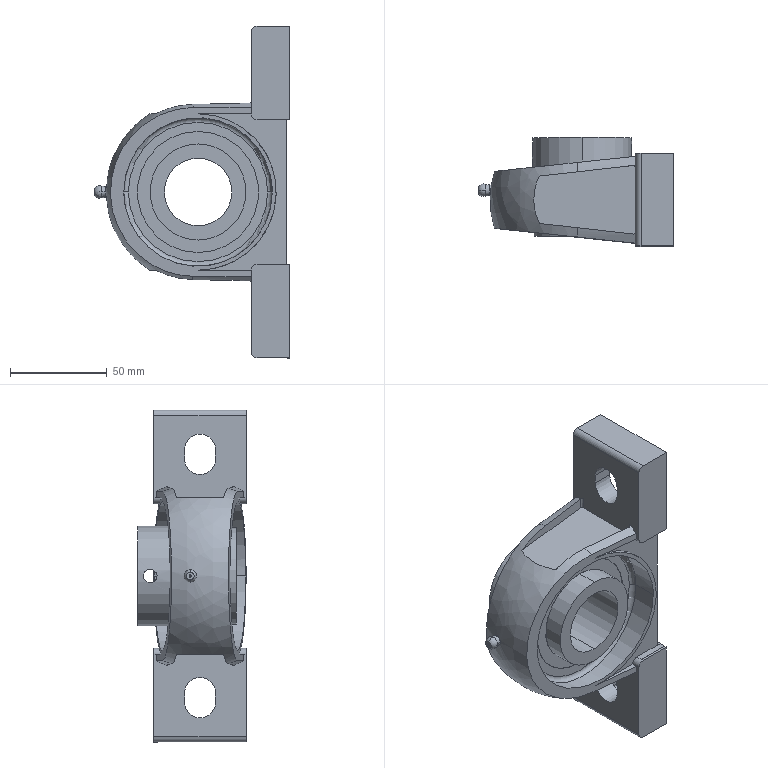Component | SolidWorks | GB_T7810-2017[BearingWithVerticalHousing(UELP)UELP207]-1 | 1 solid | 176 faces | volume 235657 mm3 | plane 67 | cylinder 46 | sphere 34 | cone 16 | torus 8 | spline 5 | commonest cylinder face diameters 2 x6 76.936 x6 62.79 x6 49.8 x6 6 x6 7.134 x4 16 x4 51.4 x2